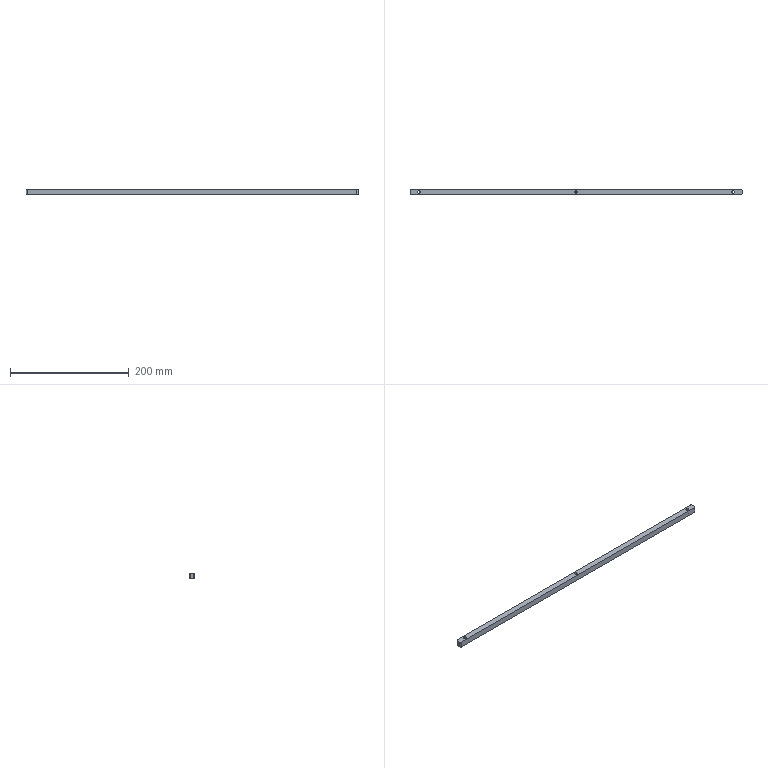Component | SolidWorks | SL010-RightStreamline-1-1_SL010-02047844SupportBar2-1-1 | 1 solid | 25 faces | box 560 x 10 x 10 mm | volume 55035 mm3 | cylinder 16 | plane 9 | commonest cylinder face diameters 8 x6 4.5 x6 4 x4 | material White POM
build123d program:
from build123d import *

# Parameters (mm, degrees)
SKETCH1_W                                       = 560
SKETCH1_H                                       = 10
BOSS_EXTRUDE1_DEPTH                             = 5
M4_HEX_SOCKET_HEAD_CAP_SCREW_CBORE1_D           = 4.5
M4_HEX_SOCKET_HEAD_CAP_SCREW_CBORE1_CBORE_D     = 8
M4_HEX_SOCKET_HEAD_CAP_SCREW_CBORE1_CBORE_DEPTH = 4.4
FILLET1_R                                       = 2


with BuildPart() as part:
    # Sketch1 → Boss-Extrude1 (new, symmetric)
    with BuildSketch(Plane.XY):
        Rectangle(SKETCH1_W, SKETCH1_H)
    extrude(amount=BOSS_EXTRUDE1_DEPTH, both=True)

    # M4 Hex Socket Head Cap Screw CBORE1 (through all)
    with Locations(Plane.XY.offset(5)):
        with Locations((-265, 0), (265, 0), (0, 0)):
            CounterBoreHole(M4_HEX_SOCKET_HEAD_CAP_SCREW_CBORE1_D / 2, M4_HEX_SOCKET_HEAD_CAP_SCREW_CBORE1_CBORE_D / 2, M4_HEX_SOCKET_HEAD_CAP_SCREW_CBORE1_CBORE_DEPTH)

    # Fillet1
    fillet1_edges = [part.edges().sort_by_distance(p)[0] for p in [
        (280, -5, 0),
        (-280, -5, 0),
        (-280, 5, 0),
        (280, 5, 0),
    ]]
    fillet(fillet1_edges, radius=FILLET1_R)


solid = part.part

# Placed as in the assembly
solid = solid.moved(Location((0, -116.404, -336.035), (180, 0, 0)))
STEP:
#1=CARTESIAN_POINT('',(10.591,-4.583,-13.253));
#2=VERTEX_POINT('',#1);
#3=CARTESIAN_POINT('',(10.276,-4.583,-13.253));
#4=VERTEX_POINT('',#3);
#5=CARTESIAN_POINT('',(10.433,-4.583,-13.253));
#6=DIRECTION('',(0.,-0.,-1.));
#7=DIRECTION('',(-1.,0.,0.));
#8=AXIS2_PLACEMENT_3D('',#5,#6,#7);
#9=CIRCLE('',#8,0.1575);
#10=EDGE_CURVE('',#2,#4,#9,.T.);
#11=ORIENTED_EDGE('',*,*,#10,.F.);
#12=CARTESIAN_POINT('',(10.591,-4.583,-13.427));
#13=VERTEX_POINT('',#12);
#14=CARTESIAN_POINT('',(10.591,-4.583,-13.427));
#15=DIRECTION('',(0.,-0.,-1.));
#16=VECTOR('',#15,39.37);
#17=LINE('',#14,#16);
#18=EDGE_CURVE('',#2,#13,#17,.T.);
#19=ORIENTED_EDGE('',*,*,#18,.T.);
#20=CARTESIAN_POINT('',(10.276,-4.583,-13.427));
#21=VERTEX_POINT('',#20);
#22=CARTESIAN_POINT('',(10.433,-4.583,-13.427));
#23=DIRECTION('',(0.,-0.,-1.));
#24=DIRECTION('',(-1.,0.,0.));
#25=AXIS2_PLACEMENT_3D('',#22,#23,#24);
#26=CIRCLE('',#25,0.1575);
#27=EDGE_CURVE('',#13,#21,#26,.T.);
#28=ORIENTED_EDGE('',*,*,#27,.T.);
#29=CARTESIAN_POINT('',(10.276,-4.583,-13.427));
#30=DIRECTION('',(0.,-0.,-1.));
#31=VECTOR('',#30,39.37);
#32=LINE('',#29,#31);
#33=EDGE_CURVE('',#4,#21,#32,.T.);
#34=ORIENTED_EDGE('',*,*,#33,.F.);
#35=EDGE_LOOP('',(#11,#19,#28,#34));
#36=FACE_OUTER_BOUND('',#35,.T.);
#37=CARTESIAN_POINT('',(10.433,-4.583,-13.427));
#38=DIRECTION('',(0.,-0.,-1.));
#39=DIRECTION('',(-1.,0.,0.));
#40=AXIS2_PLACEMENT_3D('',#37,#38,#39);
#41=CYLINDRICAL_SURFACE('',#40,0.1575);
#42=ADVANCED_FACE('',(#36),#41,.F.);
#43=CARTESIAN_POINT('',(10.522,-4.583,-13.033));
#44=VERTEX_POINT('',#43);
#45=CARTESIAN_POINT('',(10.344,-4.583,-13.033));
#46=VERTEX_POINT('',#45);
#47=CARTESIAN_POINT('',(10.433,-4.583,-13.033));
#48=DIRECTION('',(0.,-0.,-1.));
#49=DIRECTION('',(-1.,0.,0.));
#50=AXIS2_PLACEMENT_3D('',#47,#48,#49);
#51=CIRCLE('',#50,0.08858);
#52=EDGE_CURVE('',#44,#46,#51,.T.);
#53=ORIENTED_EDGE('',*,*,#52,.F.);
#54=CARTESIAN_POINT('',(10.522,-4.583,-13.253));
#55=VERTEX_POINT('',#54);
#56=CARTESIAN_POINT('',(10.522,-4.583,-13.427));
#57=DIRECTION('',(0.,-0.,-1.));
#58=VECTOR('',#57,39.37);
#59=LINE('',#56,#58);
#60=EDGE_CURVE('',#44,#55,#59,.T.);
#61=ORIENTED_EDGE('',*,*,#60,.T.);
#62=CARTESIAN_POINT('',(10.344,-4.583,-13.253));
#63=VERTEX_POINT('',#62);
#64=CARTESIAN_POINT('',(10.433,-4.583,-13.253));
#65=DIRECTION('',(0.,-0.,-1.));
#66=DIRECTION('',(-1.,0.,0.));
#67=AXIS2_PLACEMENT_3D('',#64,#65,#66);
#68=CIRCLE('',#67,0.08858);
#69=EDGE_CURVE('',#55,#63,#68,.T.);
#70=ORIENTED_EDGE('',*,*,#69,.T.);
#71=CARTESIAN_POINT('',(10.344,-4.583,-13.427));
#72=DIRECTION('',(0.,-0.,-1.));
#73=VECTOR('',#72,39.37);
#74=LINE('',#71,#73);
#75=EDGE_CURVE('',#46,#63,#74,.T.);
#76=ORIENTED_EDGE('',*,*,#75,.F.);
#77=EDGE_LOOP('',(#53,#61,#70,#76));
#78=FACE_OUTER_BOUND('',#77,.T.);
#79=CARTESIAN_POINT('',(10.433,-4.583,-13.427));
#80=DIRECTION('',(0.,-0.,-1.));
#81=DIRECTION('',(-1.,0.,0.));
#82=AXIS2_PLACEMENT_3D('',#79,#80,#81);
#83=CYLINDRICAL_SURFACE('',#82,0.08858);
#84=ADVANCED_FACE('',(#78),#83,.F.);
#85=CARTESIAN_POINT('',(-10.276,-4.583,-13.253));
#86=VERTEX_POINT('',#85);
#87=CARTESIAN_POINT('',(-10.591,-4.583,-13.253));
#88=VERTEX_POINT('',#87);
#89=CARTESIAN_POINT('',(-10.433,-4.583,-13.253));
#90=DIRECTION('',(0.,-0.,-1.));
#91=DIRECTION('',(-1.,0.,0.));
#92=AXIS2_PLACEMENT_3D('',#89,#90,#91);
#93=CIRCLE('',#92,0.1575);
#94=EDGE_CURVE('',#86,#88,#93,.T.);
#95=ORIENTED_EDGE('',*,*,#94,.F.);
#96=CARTESIAN_POINT('',(-10.276,-4.583,-13.427));
#97=VERTEX_POINT('',#96);
#98=CARTESIAN_POINT('',(-10.276,-4.583,-13.427));
#99=DIRECTION('',(0.,-0.,-1.));
#100=VECTOR('',#99,39.37);
#101=LINE('',#98,#100);
#102=EDGE_CURVE('',#86,#97,#101,.T.);
#103=ORIENTED_EDGE('',*,*,#102,.T.);
#104=CARTESIAN_POINT('',(-10.591,-4.583,-13.427));
#105=VERTEX_POINT('',#104);
#106=CARTESIAN_POINT('',(-10.433,-4.583,-13.427));
#107=DIRECTION('',(0.,-0.,-1.));
#108=DIRECTION('',(-1.,0.,0.));
#109=AXIS2_PLACEMENT_3D('',#106,#107,#108);
#110=CIRCLE('',#109,0.1575);
#111=EDGE_CURVE('',#97,#105,#110,.T.);
#112=ORIENTED_EDGE('',*,*,#111,.T.);
#113=CARTESIAN_POINT('',(-10.591,-4.583,-13.427));
#114=DIRECTION('',(0.,-0.,-1.));
#115=VECTOR('',#114,39.37);
#116=LINE('',#113,#115);
#117=EDGE_CURVE('',#88,#105,#116,.T.);
#118=ORIENTED_EDGE('',*,*,#117,.F.);
#119=EDGE_LOOP('',(#95,#103,#112,#118));
#120=FACE_OUTER_BOUND('',#119,.T.);
#121=CARTESIAN_POINT('',(-10.433,-4.583,-13.427));
#122=DIRECTION('',(0.,-0.,-1.));
#123=DIRECTION('',(-1.,0.,0.));
#124=AXIS2_PLACEMENT_3D('',#121,#122,#123);
#125=CYLINDRICAL_SURFACE('',#124,0.1575);
#126=ADVANCED_FACE('',(#120),#125,.F.);
#127=CARTESIAN_POINT('',(-10.344,-4.583,-13.033));
#128=VERTEX_POINT('',#127);
#129=CARTESIAN_POINT('',(-10.522,-4.583,-13.033));
#130=VERTEX_POINT('',#129);
#131=CARTESIAN_POINT('',(-10.433,-4.583,-13.033));
#132=DIRECTION('',(0.,-0.,-1.));
#133=DIRECTION('',(-1.,0.,0.));
#134=AXIS2_PLACEMENT_3D('',#131,#132,#133);
#135=CIRCLE('',#134,0.08858);
#136=EDGE_CURVE('',#128,#130,#135,.T.);
#137=ORIENTED_EDGE('',*,*,#136,.F.);
#138=CARTESIAN_POINT('',(-10.344,-4.583,-13.253));
#139=VERTEX_POINT('',#138);
#140=CARTESIAN_POINT('',(-10.344,-4.583,-13.427));
#141=DIRECTION('',(0.,-0.,-1.));
#142=VECTOR('',#141,39.37);
#143=LINE('',#140,#142);
#144=EDGE_CURVE('',#128,#139,#143,.T.);
#145=ORIENTED_EDGE('',*,*,#144,.T.);
#146=CARTESIAN_POINT('',(-10.522,-4.583,-13.253));
#147=VERTEX_POINT('',#146);
#148=CARTESIAN_POINT('',(-10.433,-4.583,-13.253));
#149=DIRECTION('',(0.,-0.,-1.));
#150=DIRECTION('',(-1.,0.,0.));
#151=AXIS2_PLACEMENT_3D('',#148,#149,#150);
#152=CIRCLE('',#151,0.08858);
#153=EDGE_CURVE('',#139,#147,#152,.T.);
#154=ORIENTED_EDGE('',*,*,#153,.T.);
#155=CARTESIAN_POINT('',(-10.522,-4.583,-13.427));
#156=DIRECTION('',(0.,-0.,-1.));
#157=VECTOR('',#156,39.37);
#158=LINE('',#155,#157);
#159=EDGE_CURVE('',#130,#147,#158,.T.);
#160=ORIENTED_EDGE('',*,*,#159,.F.);
#161=EDGE_LOOP('',(#137,#145,#154,#160));
#162=FACE_OUTER_BOUND('',#161,.T.);
#163=CARTESIAN_POINT('',(-10.433,-4.583,-13.427));
#164=DIRECTION('',(0.,-0.,-1.));
#165=DIRECTION('',(-1.,0.,0.));
#166=AXIS2_PLACEMENT_3D('',#163,#164,#165);
#167=CYLINDRICAL_SURFACE('',#166,0.08858);
#168=ADVANCED_FACE('',(#162),#167,.F.);
#169=CARTESIAN_POINT('',(0.1575,-4.583,-13.253));
#170=VERTEX_POINT('',#169);
#171=CARTESIAN_POINT('',(-0.1575,-4.583,-13.253));
#172=VERTEX_POINT('',#171);
#173=CARTESIAN_POINT('',(0.,-4.583,-13.253));
#174=DIRECTION('',(0.,-0.,-1.));
#175=DIRECTION('',(-1.,0.,0.));
#176=AXIS2_PLACEMENT_3D('',#173,#174,#175);
#177=CIRCLE('',#176,0.1575);
#178=EDGE_CURVE('',#170,#172,#177,.T.);
#179=ORIENTED_EDGE('',*,*,#178,.F.);
#180=CARTESIAN_POINT('',(0.1575,-4.583,-13.427));
#181=VERTEX_POINT('',#180);
#182=CARTESIAN_POINT('',(0.1575,-4.583,-13.427));
#183=DIRECTION('',(0.,-0.,-1.));
#184=VECTOR('',#183,39.37);
#185=LINE('',#182,#184);
#186=EDGE_CURVE('',#170,#181,#185,.T.);
#187=ORIENTED_EDGE('',*,*,#186,.T.);
#188=CARTESIAN_POINT('',(-0.1575,-4.583,-13.427));
#189=VERTEX_POINT('',#188);
#190=CARTESIAN_POINT('',(0.,-4.583,-13.427));
#191=DIRECTION('',(0.,-0.,-1.));
#192=DIRECTION('',(-1.,0.,0.));
#193=AXIS2_PLACEMENT_3D('',#190,#191,#192);
#194=CIRCLE('',#193,0.1575);
#195=EDGE_CURVE('',#181,#189,#194,.T.);
#196=ORIENTED_EDGE('',*,*,#195,.T.);
#197=CARTESIAN_POINT('',(-0.1575,-4.583,-13.427));
#198=DIRECTION('',(0.,-0.,-1.));
#199=VECTOR('',#198,39.37);
#200=LINE('',#197,#199);
#201=EDGE_CURVE('',#172,#189,#200,.T.);
#202=ORIENTED_EDGE('',*,*,#201,.F.);
#203=EDGE_LOOP('',(#179,#187,#196,#202));
#204=FACE_OUTER_BOUND('',#203,.T.);
#205=CARTESIAN_POINT('',(0.,-4.583,-13.427));
#206=DIRECTION('',(0.,-0.,-1.));
#207=DIRECTION('',(-1.,0.,0.));
#208=AXIS2_PLACEMENT_3D('',#205,#206,#207);
#209=CYLINDRICAL_SURFACE('',#208,0.1575);
#210=ADVANCED_FACE('',(#204),#209,.F.);
#211=CARTESIAN_POINT('',(0.08858,-4.583,-13.033));
#212=VERTEX_POINT('',#211);
#213=CARTESIAN_POINT('',(-0.08858,-4.583,-13.033));
#214=VERTEX_POINT('',#213);
#215=CARTESIAN_POINT('',(0.,-4.583,-13.033));
#216=DIRECTION('',(0.,-0.,-1.));
#217=DIRECTION('',(-1.,0.,0.));
#218=AXIS2_PLACEMENT_3D('',#215,#216,#217);
#219=CIRCLE('',#218,0.08858);
#220=EDGE_CURVE('',#212,#214,#219,.T.);
#221=ORIENTED_EDGE('',*,*,#220,.F.);
#222=CARTESIAN_POINT('',(0.08858,-4.583,-13.253));
#223=VERTEX_POINT('',#222);
#224=CARTESIAN_POINT('',(0.08858,-4.583,-13.427));
#225=DIRECTION('',(0.,-0.,-1.));
#226=VECTOR('',#225,39.37);
#227=LINE('',#224,#226);
#228=EDGE_CURVE('',#212,#223,#227,.T.);
#229=ORIENTED_EDGE('',*,*,#228,.T.);
#230=CARTESIAN_POINT('',(-0.08858,-4.583,-13.253));
#231=VERTEX_POINT('',#230);
#232=CARTESIAN_POINT('',(0.,-4.583,-13.253));
#233=DIRECTION('',(0.,-0.,-1.));
#234=DIRECTION('',(-1.,0.,0.));
#235=AXIS2_PLACEMENT_3D('',#232,#233,#234);
#236=CIRCLE('',#235,0.08858);
#237=EDGE_CURVE('',#223,#231,#236,.T.);
#238=ORIENTED_EDGE('',*,*,#237,.T.);
#239=CARTESIAN_POINT('',(-0.08858,-4.583,-13.427));
#240=DIRECTION('',(0.,-0.,-1.));
#241=VECTOR('',#240,39.37);
#242=LINE('',#239,#241);
#243=EDGE_CURVE('',#214,#231,#242,.T.);
#244=ORIENTED_EDGE('',*,*,#243,.F.);
#245=EDGE_LOOP('',(#221,#229,#238,#244));
#246=FACE_OUTER_BOUND('',#245,.T.);
#247=CARTESIAN_POINT('',(0.,-4.583,-13.427));
#248=DIRECTION('',(0.,-0.,-1.));
#249=DIRECTION('',(-1.,0.,0.));
#250=AXIS2_PLACEMENT_3D('',#247,#248,#249);
#251=CYLINDRICAL_SURFACE('',#250,0.08858);
#252=ADVANCED_FACE('',(#246),#251,.F.);
#253=CARTESIAN_POINT('',(-11.024,-4.701,-13.427));
#254=VERTEX_POINT('',#253);
#255=CARTESIAN_POINT('',(-11.024,-4.465,-13.427));
#256=VERTEX_POINT('',#255);
#257=CARTESIAN_POINT('',(-11.024,-4.386,-13.427));
#258=DIRECTION('',(0.,1.,-0.));
#259=VECTOR('',#258,39.37);
#260=LINE('',#257,#259);
#261=EDGE_CURVE('',#254,#256,#260,.T.);
#262=ORIENTED_EDGE('',*,*,#261,.F.);
#263=CARTESIAN_POINT('',(-11.024,-4.701,-13.033));
#264=VERTEX_POINT('',#263);
#265=CARTESIAN_POINT('',(-11.024,-4.701,-13.427));
#266=DIRECTION('',(-0.,0.,1.));
#267=VECTOR('',#266,39.37);
#268=LINE('',#265,#267);
#269=EDGE_CURVE('',#254,#264,#268,.T.);
#270=ORIENTED_EDGE('',*,*,#269,.T.);
#271=CARTESIAN_POINT('',(-11.024,-4.465,-13.033));
#272=VERTEX_POINT('',#271);
#273=CARTESIAN_POINT('',(-11.024,-4.386,-13.033));
#274=DIRECTION('',(0.,1.,-0.));
#275=VECTOR('',#274,39.37);
#276=LINE('',#273,#275);
#277=EDGE_CURVE('',#264,#272,#276,.T.);
#278=ORIENTED_EDGE('',*,*,#277,.T.);
#279=CARTESIAN_POINT('',(-11.024,-4.465,-13.427));
#280=DIRECTION('',(0.,-0.,-1.));
#281=VECTOR('',#280,39.37);
#282=LINE('',#279,#281);
#283=EDGE_CURVE('',#272,#256,#282,.T.);
#284=ORIENTED_EDGE('',*,*,#283,.T.);
#285=EDGE_LOOP('',(#262,#270,#278,#284));
#286=FACE_OUTER_BOUND('',#285,.T.);
#287=CARTESIAN_POINT('',(-11.024,-4.386,-13.427));
#288=DIRECTION('',(1.,0.,0.));
#289=DIRECTION('',(0.,-0.,-1.));
#290=AXIS2_PLACEMENT_3D('',#287,#288,#289);
#291=PLANE('',#290);
#292=ADVANCED_FACE('',(#286),#291,.F.);
#293=CARTESIAN_POINT('',(-10.945,-4.386,-13.427));
#294=VERTEX_POINT('',#293);
#295=CARTESIAN_POINT('',(10.945,-4.386,-13.427));
#296=VERTEX_POINT('',#295);
#297=CARTESIAN_POINT('',(11.024,-4.386,-13.427));
#298=DIRECTION('',(1.,0.,-0.));
#299=VECTOR('',#298,39.37);
#300=LINE('',#297,#299);
#301=EDGE_CURVE('',#294,#296,#300,.T.);
#302=ORIENTED_EDGE('',*,*,#301,.F.);
#303=CARTESIAN_POINT('',(-10.945,-4.386,-13.033));
#304=VERTEX_POINT('',#303);
#305=CARTESIAN_POINT('',(-10.945,-4.386,-13.427));
#306=DIRECTION('',(-0.,0.,1.));
#307=VECTOR('',#306,39.37);
#308=LINE('',#305,#307);
#309=EDGE_CURVE('',#294,#304,#308,.T.);
#310=ORIENTED_EDGE('',*,*,#309,.T.);
#311=CARTESIAN_POINT('',(10.945,-4.386,-13.033));
#312=VERTEX_POINT('',#311);
#313=CARTESIAN_POINT('',(11.024,-4.386,-13.033));
#314=DIRECTION('',(1.,0.,-0.));
#315=VECTOR('',#314,39.37);
#316=LINE('',#313,#315);
#317=EDGE_CURVE('',#304,#312,#316,.T.);
#318=ORIENTED_EDGE('',*,*,#317,.T.);
#319=CARTESIAN_POINT('',(10.945,-4.386,-13.427));
#320=DIRECTION('',(0.,-0.,-1.));
#321=VECTOR('',#320,39.37);
#322=LINE('',#319,#321);
#323=EDGE_CURVE('',#312,#296,#322,.T.);
#324=ORIENTED_EDGE('',*,*,#323,.T.);
#325=EDGE_LOOP('',(#302,#310,#318,#324));
#326=FACE_OUTER_BOUND('',#325,.T.);
#327=CARTESIAN_POINT('',(11.024,-4.386,-13.427));
#328=DIRECTION('',(-0.,-1.,0.));
#329=DIRECTION('',(-0.,0.,1.));
#330=AXIS2_PLACEMENT_3D('',#327,#328,#329);
#331=PLANE('',#330);
#332=ADVANCED_FACE('',(#326),#331,.F.);
#333=CARTESIAN_POINT('',(11.024,-4.465,-13.033));
#334=VERTEX_POINT('',#333);
#335=CARTESIAN_POINT('',(11.024,-4.701,-13.033));
#336=VERTEX_POINT('',#335);
#337=CARTESIAN_POINT('',(11.024,-4.386,-13.033));
#338=DIRECTION('',(-0.,-1.,0.));
#339=VECTOR('',#338,39.37);
#340=LINE('',#337,#339);
#341=EDGE_CURVE('',#334,#336,#340,.T.);
#342=ORIENTED_EDGE('',*,*,#341,.T.);
#343=CARTESIAN_POINT('',(11.024,-4.701,-13.427));
#344=VERTEX_POINT('',#343);
#345=CARTESIAN_POINT('',(11.024,-4.701,-13.427));
#346=DIRECTION('',(0.,-0.,-1.));
#347=VECTOR('',#346,39.37);
#348=LINE('',#345,#347);
#349=EDGE_CURVE('',#336,#344,#348,.T.);
#350=ORIENTED_EDGE('',*,*,#349,.T.);
#351=CARTESIAN_POINT('',(11.024,-4.465,-13.427));
#352=VERTEX_POINT('',#351);
#353=CARTESIAN_POINT('',(11.024,-4.386,-13.427));
#354=DIRECTION('',(-0.,-1.,0.));
#355=VECTOR('',#354,39.37);
#356=LINE('',#353,#355);
#357=EDGE_CURVE('',#352,#344,#356,.T.);
#358=ORIENTED_EDGE('',*,*,#357,.F.);
#359=CARTESIAN_POINT('',(11.024,-4.465,-13.427));
#360=DIRECTION('',(-0.,0.,1.));
#361=VECTOR('',#360,39.37);
#362=LINE('',#359,#361);
#363=EDGE_CURVE('',#352,#334,#362,.T.);
#364=ORIENTED_EDGE('',*,*,#363,.T.);
#365=EDGE_LOOP('',(#342,#350,#358,#364));
#366=FACE_OUTER_BOUND('',#365,.T.);
#367=CARTESIAN_POINT('',(11.024,-4.386,-13.427));
#368=DIRECTION('',(-1.,-0.,-0.));
#369=DIRECTION('',(-0.,0.,1.));
#370=AXIS2_PLACEMENT_3D('',#367,#368,#369);
#371=PLANE('',#370);
#372=ADVANCED_FACE('',(#366),#371,.F.);
#373=CARTESIAN_POINT('',(10.945,-4.78,-13.033));
#374=VERTEX_POINT('',#373);
#375=CARTESIAN_POINT('',(-10.945,-4.78,-13.033));
#376=VERTEX_POINT('',#375);
#377=CARTESIAN_POINT('',(11.024,-4.78,-13.033));
#378=DIRECTION('',(-1.,-0.,0.));
#379=VECTOR('',#378,39.37);
#380=LINE('',#377,#379);
#381=EDGE_CURVE('',#374,#376,#380,.T.);
#382=ORIENTED_EDGE('',*,*,#381,.T.);
#383=CARTESIAN_POINT('',(-10.945,-4.78,-13.427));
#384=VERTEX_POINT('',#383);
#385=CARTESIAN_POINT('',(-10.945,-4.78,-13.427));
#386=DIRECTION('',(0.,-0.,-1.));
#387=VECTOR('',#386,39.37);
#388=LINE('',#385,#387);
#389=EDGE_CURVE('',#376,#384,#388,.T.);
#390=ORIENTED_EDGE('',*,*,#389,.T.);
#391=CARTESIAN_POINT('',(10.945,-4.78,-13.427));
#392=VERTEX_POINT('',#391);
#393=CARTESIAN_POINT('',(11.024,-4.78,-13.427));
#394=DIRECTION('',(-1.,-0.,0.));
#395=VECTOR('',#394,39.37);
#396=LINE('',#393,#395);
#397=EDGE_CURVE('',#392,#384,#396,.T.);
#398=ORIENTED_EDGE('',*,*,#397,.F.);
#399=CARTESIAN_POINT('',(10.945,-4.78,-13.427));
#400=DIRECTION('',(-0.,0.,1.));
#401=VECTOR('',#400,39.37);
#402=LINE('',#399,#401);
#403=EDGE_CURVE('',#392,#374,#402,.T.);
#404=ORIENTED_EDGE('',*,*,#403,.T.);
#405=EDGE_LOOP('',(#382,#390,#398,#404));
#406=FACE_OUTER_BOUND('',#405,.T.);
#407=CARTESIAN_POINT('',(11.024,-4.78,-13.427));
#408=DIRECTION('',(0.,1.,-0.));
#409=DIRECTION('',(0.,-0.,-1.));
#410=AXIS2_PLACEMENT_3D('',#407,#408,#409);
#411=PLANE('',#410);
#412=ADVANCED_FACE('',(#406),#411,.F.);
#413=CARTESIAN_POINT('',(10.433,-4.583,-13.427));
#414=DIRECTION('',(0.,-0.,-1.));
#415=DIRECTION('',(-1.,0.,0.));
#416=AXIS2_PLACEMENT_3D('',#413,#414,#415);
#417=CIRCLE('',#416,0.1575);
#418=EDGE_CURVE('',#21,#13,#417,.T.);
#419=ORIENTED_EDGE('',*,*,#418,.F.);
#420=ORIENTED_EDGE('',*,*,#27,.F.);
#421=EDGE_LOOP('',(#419,#420));
#422=FACE_BOUND('',#421,.T.);
#423=CARTESIAN_POINT('',(-10.433,-4.583,-13.427));
#424=DIRECTION('',(0.,-0.,-1.));
#425=DIRECTION('',(-1.,0.,0.));
#426=AXIS2_PLACEMENT_3D('',#423,#424,#425);
#427=CIRCLE('',#426,0.1575);
#428=EDGE_CURVE('',#105,#97,#427,.T.);
#429=ORIENTED_EDGE('',*,*,#428,.F.);
#430=ORIENTED_EDGE('',*,*,#111,.F.);
#431=EDGE_LOOP('',(#429,#430));
#432=FACE_BOUND('',#431,.T.);
#433=CARTESIAN_POINT('',(0.,-4.583,-13.427));
#434=DIRECTION('',(0.,-0.,-1.));
#435=DIRECTION('',(-1.,0.,0.));
#436=AXIS2_PLACEMENT_3D('',#433,#434,#435);
#437=CIRCLE('',#436,0.1575);
#438=EDGE_CURVE('',#189,#181,#437,.T.);
#439=ORIENTED_EDGE('',*,*,#438,.F.);
#440=ORIENTED_EDGE('',*,*,#195,.F.);
#441=EDGE_LOOP('',(#439,#440));
#442=FACE_BOUND('',#441,.T.);
#443=ORIENTED_EDGE('',*,*,#397,.T.);
#444=CARTESIAN_POINT('',(-10.945,-4.701,-13.427));
#445=DIRECTION('',(0.,-0.,-1.));
#446=DIRECTION('',(-1.,0.,0.));
#447=AXIS2_PLACEMENT_3D('',#444,#445,#446);
#448=CIRCLE('',#447,0.07874);
#449=EDGE_CURVE('',#384,#254,#448,.T.);
#450=ORIENTED_EDGE('',*,*,#449,.T.);
#451=ORIENTED_EDGE('',*,*,#261,.T.);
#452=CARTESIAN_POINT('',(-10.945,-4.465,-13.427));
#453=DIRECTION('',(0.,-0.,-1.));
#454=DIRECTION('',(-1.,0.,0.));
#455=AXIS2_PLACEMENT_3D('',#452,#453,#454);
#456=CIRCLE('',#455,0.07874);
#457=EDGE_CURVE('',#256,#294,#456,.T.);
#458=ORIENTED_EDGE('',*,*,#457,.T.);
#459=ORIENTED_EDGE('',*,*,#301,.T.);
#460=CARTESIAN_POINT('',(10.945,-4.465,-13.427));
#461=DIRECTION('',(0.,-0.,-1.));
#462=DIRECTION('',(-1.,0.,0.));
#463=AXIS2_PLACEMENT_3D('',#460,#461,#462);
#464=CIRCLE('',#463,0.07874);
#465=EDGE_CURVE('',#296,#352,#464,.T.);
#466=ORIENTED_EDGE('',*,*,#465,.T.);
#467=ORIENTED_EDGE('',*,*,#357,.T.);
#468=CARTESIAN_POINT('',(10.945,-4.701,-13.427));
#469=DIRECTION('',(0.,-0.,-1.));
#470=DIRECTION('',(-1.,0.,0.));
#471=AXIS2_PLACEMENT_3D('',#468,#469,#470);
#472=CIRCLE('',#471,0.07874);
#473=EDGE_CURVE('',#344,#392,#472,.T.);
#474=ORIENTED_EDGE('',*,*,#473,.T.);
#475=EDGE_LOOP('',(#443,#450,#451,#458,#459,#466,#467,#474));
#476=FACE_OUTER_BOUND('',#475,.T.);
#477=CARTESIAN_POINT('',(0.,-4.583,-13.427));
#478=DIRECTION('',(-0.,-0.,-1.));
#479=DIRECTION('',(-1.,-0.,0.));
#480=AXIS2_PLACEMENT_3D('',#477,#478,#479);
#481=PLANE('',#480);
#482=ADVANCED_FACE('',(#422,#432,#442,#476),#481,.T.);
#483=CARTESIAN_POINT('',(10.433,-4.583,-13.033));
#484=DIRECTION('',(0.,-0.,-1.));
#485=DIRECTION('',(-1.,0.,0.));
#486=AXIS2_PLACEMENT_3D('',#483,#484,#485);
#487=CIRCLE('',#486,0.08858);
#488=EDGE_CURVE('',#46,#44,#487,.T.);
#489=ORIENTED_EDGE('',*,*,#488,.T.);
#490=ORIENTED_EDGE('',*,*,#52,.T.);
#491=EDGE_LOOP('',(#489,#490));
#492=FACE_BOUND('',#491,.T.);
#493=CARTESIAN_POINT('',(-10.433,-4.583,-13.033));
#494=DIRECTION('',(0.,-0.,-1.));
#495=DIRECTION('',(-1.,0.,0.));
#496=AXIS2_PLACEMENT_3D('',#493,#494,#495);
#497=CIRCLE('',#496,0.08858);
#498=EDGE_CURVE('',#130,#128,#497,.T.);
#499=ORIENTED_EDGE('',*,*,#498,.T.);
#500=ORIENTED_EDGE('',*,*,#136,.T.);
#501=EDGE_LOOP('',(#499,#500));
#502=FACE_BOUND('',#501,.T.);
#503=CARTESIAN_POINT('',(0.,-4.583,-13.033));
#504=DIRECTION('',(0.,-0.,-1.));
#505=DIRECTION('',(-1.,0.,0.));
#506=AXIS2_PLACEMENT_3D('',#503,#504,#505);
#507=CIRCLE('',#506,0.08858);
#508=EDGE_CURVE('',#214,#212,#507,.T.);
#509=ORIENTED_EDGE('',*,*,#508,.T.);
#510=ORIENTED_EDGE('',*,*,#220,.T.);
#511=EDGE_LOOP('',(#509,#510));
#512=FACE_BOUND('',#511,.T.);
#513=ORIENTED_EDGE('',*,*,#277,.F.);
#514=CARTESIAN_POINT('',(-10.945,-4.701,-13.033));
#515=DIRECTION('',(-0.,0.,1.));
#516=DIRECTION('',(-1.,0.,0.));
#517=AXIS2_PLACEMENT_3D('',#514,#515,#516);
#518=CIRCLE('',#517,0.07874);
#519=EDGE_CURVE('',#264,#376,#518,.T.);
#520=ORIENTED_EDGE('',*,*,#519,.T.);
#521=ORIENTED_EDGE('',*,*,#381,.F.);
#522=CARTESIAN_POINT('',(10.945,-4.701,-13.033));
#523=DIRECTION('',(-0.,0.,1.));
#524=DIRECTION('',(-1.,0.,0.));
#525=AXIS2_PLACEMENT_3D('',#522,#523,#524);
#526=CIRCLE('',#525,0.07874);
#527=EDGE_CURVE('',#374,#336,#526,.T.);
#528=ORIENTED_EDGE('',*,*,#527,.T.);
#529=ORIENTED_EDGE('',*,*,#341,.F.);
#530=CARTESIAN_POINT('',(10.945,-4.465,-13.033));
#531=DIRECTION('',(-0.,0.,1.));
#532=DIRECTION('',(-1.,0.,0.));
#533=AXIS2_PLACEMENT_3D('',#530,#531,#532);
#534=CIRCLE('',#533,0.07874);
#535=EDGE_CURVE('',#334,#312,#534,.T.);
#536=ORIENTED_EDGE('',*,*,#535,.T.);
#537=ORIENTED_EDGE('',*,*,#317,.F.);
#538=CARTESIAN_POINT('',(-10.945,-4.465,-13.033));
#539=DIRECTION('',(-0.,0.,1.));
#540=DIRECTION('',(-1.,0.,0.));
#541=AXIS2_PLACEMENT_3D('',#538,#539,#540);
#542=CIRCLE('',#541,0.07874);
#543=EDGE_CURVE('',#304,#272,#542,.T.);
#544=ORIENTED_EDGE('',*,*,#543,.T.);
#545=EDGE_LOOP('',(#513,#520,#521,#528,#529,#536,#537,#544));
#546=FACE_OUTER_BOUND('',#545,.T.);
#547=CARTESIAN_POINT('',(0.,-4.583,-13.033));
#548=DIRECTION('',(-0.,-0.,-1.));
#549=DIRECTION('',(-1.,-0.,0.));
#550=AXIS2_PLACEMENT_3D('',#547,#548,#549);
#551=PLANE('',#550);
#552=ADVANCED_FACE('',(#492,#502,#512,#546),#551,.F.);
#553=ORIENTED_EDGE('',*,*,#228,.F.);
#554=ORIENTED_EDGE('',*,*,#508,.F.);
#555=ORIENTED_EDGE('',*,*,#243,.T.);
#556=CARTESIAN_POINT('',(0.,-4.583,-13.253));
#557=DIRECTION('',(0.,-0.,-1.));
#558=DIRECTION('',(-1.,0.,0.));
#559=AXIS2_PLACEMENT_3D('',#556,#557,#558);
#560=CIRCLE('',#559,0.08858);
#561=EDGE_CURVE('',#231,#223,#560,.T.);
#562=ORIENTED_EDGE('',*,*,#561,.T.);
#563=EDGE_LOOP('',(#553,#554,#555,#562));
#564=FACE_OUTER_BOUND('',#563,.T.);
#565=CARTESIAN_POINT('',(0.,-4.583,-13.427));
#566=DIRECTION('',(0.,-0.,-1.));
#567=DIRECTION('',(-1.,0.,0.));
#568=AXIS2_PLACEMENT_3D('',#565,#566,#567);
#569=CYLINDRICAL_SURFACE('',#568,0.08858);
#570=ADVANCED_FACE('',(#564),#569,.F.);
#571=ORIENTED_EDGE('',*,*,#561,.F.);
#572=ORIENTED_EDGE('',*,*,#237,.F.);
#573=EDGE_LOOP('',(#571,#572));
#574=FACE_BOUND('',#573,.T.);
#575=CARTESIAN_POINT('',(0.,-4.583,-13.253));
#576=DIRECTION('',(0.,-0.,-1.));
#577=DIRECTION('',(-1.,0.,0.));
#578=AXIS2_PLACEMENT_3D('',#575,#576,#577);
#579=CIRCLE('',#578,0.1575);
#580=EDGE_CURVE('',#172,#170,#579,.T.);
#581=ORIENTED_EDGE('',*,*,#580,.T.);
#582=ORIENTED_EDGE('',*,*,#178,.T.);
#583=EDGE_LOOP('',(#581,#582));
#584=FACE_OUTER_BOUND('',#583,.T.);
#585=CARTESIAN_POINT('',(-0.08858,-4.583,-13.253));
#586=DIRECTION('',(0.,0.,1.));
#587=DIRECTION('',(1.,0.,-0.));
#588=AXIS2_PLACEMENT_3D('',#585,#586,#587);
#589=PLANE('',#588);
#590=ADVANCED_FACE('',(#574,#584),#589,.F.);
#591=ORIENTED_EDGE('',*,*,#186,.F.);
#592=ORIENTED_EDGE('',*,*,#580,.F.);
#593=ORIENTED_EDGE('',*,*,#201,.T.);
#594=ORIENTED_EDGE('',*,*,#438,.T.);
#595=EDGE_LOOP('',(#591,#592,#593,#594));
#596=FACE_OUTER_BOUND('',#595,.T.);
#597=CARTESIAN_POINT('',(0.,-4.583,-13.427));
#598=DIRECTION('',(0.,-0.,-1.));
#599=DIRECTION('',(-1.,0.,0.));
#600=AXIS2_PLACEMENT_3D('',#597,#598,#599);
#601=CYLINDRICAL_SURFACE('',#600,0.1575);
#602=ADVANCED_FACE('',(#596),#601,.F.);
#603=ORIENTED_EDGE('',*,*,#144,.F.);
#604=ORIENTED_EDGE('',*,*,#498,.F.);
#605=ORIENTED_EDGE('',*,*,#159,.T.);
#606=CARTESIAN_POINT('',(-10.433,-4.583,-13.253));
#607=DIRECTION('',(0.,-0.,-1.));
#608=DIRECTION('',(-1.,0.,0.));
#609=AXIS2_PLACEMENT_3D('',#606,#607,#608);
#610=CIRCLE('',#609,0.08858);
#611=EDGE_CURVE('',#147,#139,#610,.T.);
#612=ORIENTED_EDGE('',*,*,#611,.T.);
#613=EDGE_LOOP('',(#603,#604,#605,#612));
#614=FACE_OUTER_BOUND('',#613,.T.);
#615=CARTESIAN_POINT('',(-10.433,-4.583,-13.427));
#616=DIRECTION('',(0.,-0.,-1.));
#617=DIRECTION('',(-1.,0.,0.));
#618=AXIS2_PLACEMENT_3D('',#615,#616,#617);
#619=CYLINDRICAL_SURFACE('',#618,0.08858);
#620=ADVANCED_FACE('',(#614),#619,.F.);
#621=ORIENTED_EDGE('',*,*,#611,.F.);
#622=ORIENTED_EDGE('',*,*,#153,.F.);
#623=EDGE_LOOP('',(#621,#622));
#624=FACE_BOUND('',#623,.T.);
#625=CARTESIAN_POINT('',(-10.433,-4.583,-13.253));
#626=DIRECTION('',(0.,-0.,-1.));
#627=DIRECTION('',(-1.,0.,0.));
#628=AXIS2_PLACEMENT_3D('',#625,#626,#627);
#629=CIRCLE('',#628,0.1575);
#630=EDGE_CURVE('',#88,#86,#629,.T.);
#631=ORIENTED_EDGE('',*,*,#630,.T.);
#632=ORIENTED_EDGE('',*,*,#94,.T.);
#633=EDGE_LOOP('',(#631,#632));
#634=FACE_OUTER_BOUND('',#633,.T.);
#635=CARTESIAN_POINT('',(-10.522,-4.583,-13.253));
#636=DIRECTION('',(0.,0.,1.));
#637=DIRECTION('',(1.,0.,-0.));
#638=AXIS2_PLACEMENT_3D('',#635,#636,#637);
#639=PLANE('',#638);
#640=ADVANCED_FACE('',(#624,#634),#639,.F.);
#641=ORIENTED_EDGE('',*,*,#102,.F.);
#642=ORIENTED_EDGE('',*,*,#630,.F.);
#643=ORIENTED_EDGE('',*,*,#117,.T.);
#644=ORIENTED_EDGE('',*,*,#428,.T.);
#645=EDGE_LOOP('',(#641,#642,#643,#644));
#646=FACE_OUTER_BOUND('',#645,.T.);
#647=CARTESIAN_POINT('',(-10.433,-4.583,-13.427));
#648=DIRECTION('',(0.,-0.,-1.));
#649=DIRECTION('',(-1.,0.,0.));
#650=AXIS2_PLACEMENT_3D('',#647,#648,#649);
#651=CYLINDRICAL_SURFACE('',#650,0.1575);
#652=ADVANCED_FACE('',(#646),#651,.F.);
#653=ORIENTED_EDGE('',*,*,#60,.F.);
#654=ORIENTED_EDGE('',*,*,#488,.F.);
#655=ORIENTED_EDGE('',*,*,#75,.T.);
#656=CARTESIAN_POINT('',(10.433,-4.583,-13.253));
#657=DIRECTION('',(0.,-0.,-1.));
#658=DIRECTION('',(-1.,0.,0.));
#659=AXIS2_PLACEMENT_3D('',#656,#657,#658);
#660=CIRCLE('',#659,0.08858);
#661=EDGE_CURVE('',#63,#55,#660,.T.);
#662=ORIENTED_EDGE('',*,*,#661,.T.);
#663=EDGE_LOOP('',(#653,#654,#655,#662));
#664=FACE_OUTER_BOUND('',#663,.T.);
#665=CARTESIAN_POINT('',(10.433,-4.583,-13.427));
#666=DIRECTION('',(0.,-0.,-1.));
#667=DIRECTION('',(-1.,0.,0.));
#668=AXIS2_PLACEMENT_3D('',#665,#666,#667);
#669=CYLINDRICAL_SURFACE('',#668,0.08858);
#670=ADVANCED_FACE('',(#664),#669,.F.);
#671=ORIENTED_EDGE('',*,*,#661,.F.);
#672=ORIENTED_EDGE('',*,*,#69,.F.);
#673=EDGE_LOOP('',(#671,#672));
#674=FACE_BOUND('',#673,.T.);
#675=CARTESIAN_POINT('',(10.433,-4.583,-13.253));
#676=DIRECTION('',(0.,-0.,-1.));
#677=DIRECTION('',(-1.,0.,0.));
#678=AXIS2_PLACEMENT_3D('',#675,#676,#677);
#679=CIRCLE('',#678,0.1575);
#680=EDGE_CURVE('',#4,#2,#679,.T.);
#681=ORIENTED_EDGE('',*,*,#680,.T.);
#682=ORIENTED_EDGE('',*,*,#10,.T.);
#683=EDGE_LOOP('',(#681,#682));
#684=FACE_OUTER_BOUND('',#683,.T.);
#685=CARTESIAN_POINT('',(10.344,-4.583,-13.253));
#686=DIRECTION('',(0.,0.,1.));
#687=DIRECTION('',(1.,0.,-0.));
#688=AXIS2_PLACEMENT_3D('',#685,#686,#687);
#689=PLANE('',#688);
#690=ADVANCED_FACE('',(#674,#684),#689,.F.);
#691=ORIENTED_EDGE('',*,*,#18,.F.);
#692=ORIENTED_EDGE('',*,*,#680,.F.);
#693=ORIENTED_EDGE('',*,*,#33,.T.);
#694=ORIENTED_EDGE('',*,*,#418,.T.);
#695=EDGE_LOOP('',(#691,#692,#693,#694));
#696=FACE_OUTER_BOUND('',#695,.T.);
#697=CARTESIAN_POINT('',(10.433,-4.583,-13.427));
#698=DIRECTION('',(0.,-0.,-1.));
#699=DIRECTION('',(-1.,0.,0.));
#700=AXIS2_PLACEMENT_3D('',#697,#698,#699);
#701=CYLINDRICAL_SURFACE('',#700,0.1575);
#702=ADVANCED_FACE('',(#696),#701,.F.);
#703=ORIENTED_EDGE('',*,*,#449,.F.);
#704=ORIENTED_EDGE('',*,*,#389,.F.);
#705=ORIENTED_EDGE('',*,*,#519,.F.);
#706=ORIENTED_EDGE('',*,*,#269,.F.);
#707=EDGE_LOOP('',(#703,#704,#705,#706));
#708=FACE_OUTER_BOUND('',#707,.T.);
#709=CARTESIAN_POINT('',(-10.945,-4.701,-13.427));
#710=DIRECTION('',(-0.,0.,1.));
#711=DIRECTION('',(1.,0.,0.));
#712=AXIS2_PLACEMENT_3D('',#709,#710,#711);
#713=CYLINDRICAL_SURFACE('',#712,0.07874);
#714=ADVANCED_FACE('',(#708),#713,.T.);
#715=ORIENTED_EDGE('',*,*,#457,.F.);
#716=ORIENTED_EDGE('',*,*,#283,.F.);
#717=ORIENTED_EDGE('',*,*,#543,.F.);
#718=ORIENTED_EDGE('',*,*,#309,.F.);
#719=EDGE_LOOP('',(#715,#716,#717,#718));
#720=FACE_OUTER_BOUND('',#719,.T.);
#721=CARTESIAN_POINT('',(-10.945,-4.465,-13.427));
#722=DIRECTION('',(-0.,0.,1.));
#723=DIRECTION('',(1.,0.,0.));
#724=AXIS2_PLACEMENT_3D('',#721,#722,#723);
#725=CYLINDRICAL_SURFACE('',#724,0.07874);
#726=ADVANCED_FACE('',(#720),#725,.T.);
#727=ORIENTED_EDGE('',*,*,#473,.F.);
#728=ORIENTED_EDGE('',*,*,#349,.F.);
#729=ORIENTED_EDGE('',*,*,#527,.F.);
#730=ORIENTED_EDGE('',*,*,#403,.F.);
#731=EDGE_LOOP('',(#727,#728,#729,#730));
#732=FACE_OUTER_BOUND('',#731,.T.);
#733=CARTESIAN_POINT('',(10.945,-4.701,-13.427));
#734=DIRECTION('',(-0.,0.,1.));
#735=DIRECTION('',(1.,0.,0.));
#736=AXIS2_PLACEMENT_3D('',#733,#734,#735);
#737=CYLINDRICAL_SURFACE('',#736,0.07874);
#738=ADVANCED_FACE('',(#732),#737,.T.);
#739=ORIENTED_EDGE('',*,*,#465,.F.);
#740=ORIENTED_EDGE('',*,*,#323,.F.);
#741=ORIENTED_EDGE('',*,*,#535,.F.);
#742=ORIENTED_EDGE('',*,*,#363,.F.);
#743=EDGE_LOOP('',(#739,#740,#741,#742));
#744=FACE_OUTER_BOUND('',#743,.T.);
#745=CARTESIAN_POINT('',(10.945,-4.465,-13.427));
#746=DIRECTION('',(-0.,0.,1.));
#747=DIRECTION('',(1.,0.,0.));
#748=AXIS2_PLACEMENT_3D('',#745,#746,#747);
#749=CYLINDRICAL_SURFACE('',#748,0.07874);
#750=ADVANCED_FACE('',(#744),#749,.T.);
#751=CLOSED_SHELL('',(#42,#84,#126,#168,#210,#252,#292,#332,#372,#412,#482,#552,#570,#590,#602,#620,#640,#652,#670,#690,#702,#714,#726,#738,#750));
#752=MANIFOLD_SOLID_BREP('',#751);
#753=CARTESIAN_POINT('',(0.,0.,0.));
#754=DIRECTION('',(0.,0.,1.));
#755=DIRECTION('',(1.,0.,0.));
#756=AXIS2_PLACEMENT_3D('',#753,#754,#755);
#757=(LENGTH_UNIT()NAMED_UNIT(*)SI_UNIT($,.METRE.));
#758=LENGTH_MEASURE_WITH_UNIT(LENGTH_MEASURE(0.0254),#757);
#759=DIMENSIONAL_EXPONENTS(1.,0.,0.,0.,0.,0.,0.);
#760=(CONVERSION_BASED_UNIT('',#758)LENGTH_UNIT()NAMED_UNIT(#759));
#761=UNCERTAINTY_MEASURE_WITH_UNIT(LENGTH_MEASURE(0.00001),#760,'','');
#762=(NAMED_UNIT(*)PLANE_ANGLE_UNIT()SI_UNIT($,.RADIAN.));
#763=(NAMED_UNIT(*)SI_UNIT($,.STERADIAN.)SOLID_ANGLE_UNIT());
#764=(GEOMETRIC_REPRESENTATION_CONTEXT(3)GLOBAL_UNCERTAINTY_ASSIGNED_CONTEXT((#761))GLOBAL_UNIT_ASSIGNED_CONTEXT((#760,#762,#763))REPRESENTATION_CONTEXT('',''));
#765=ADVANCED_BREP_SHAPE_REPRESENTATION('',(#752,#756),#764);
#766=COLOUR_RGB('',0.7922,0.8196,0.9333);
#767=FILL_AREA_STYLE_COLOUR('',#766);
#768=FILL_AREA_STYLE('',(#767));
#769=SURFACE_STYLE_FILL_AREA(#768);
#770=SURFACE_SIDE_STYLE('',(#769));
#771=SURFACE_STYLE_USAGE(.BOTH.,#770);
#772=PRESENTATION_STYLE_ASSIGNMENT((#771));
#773=STYLED_ITEM('',(#772),#752);
#774=PRESENTATION_LAYER_ASSIGNMENT('','',(#773));
#775=(LENGTH_UNIT()NAMED_UNIT(*)SI_UNIT($,.METRE.));
#776=LENGTH_MEASURE_WITH_UNIT(LENGTH_MEASURE(0.0254),#775);
#777=DIMENSIONAL_EXPONENTS(1.,0.,0.,0.,0.,0.,0.);
#778=(CONVERSION_BASED_UNIT('',#776)LENGTH_UNIT()NAMED_UNIT(#777));
#779=UNCERTAINTY_MEASURE_WITH_UNIT(LENGTH_MEASURE(0.00001),#778,'','');
#780=(NAMED_UNIT(*)PLANE_ANGLE_UNIT()SI_UNIT($,.RADIAN.));
#781=(NAMED_UNIT(*)SI_UNIT($,.STERADIAN.)SOLID_ANGLE_UNIT());
#782=(GEOMETRIC_REPRESENTATION_CONTEXT(3)GLOBAL_UNCERTAINTY_ASSIGNED_CONTEXT((#779))GLOBAL_UNIT_ASSIGNED_CONTEXT((#778,#780,#781))REPRESENTATION_CONTEXT('',''));
#783=MECHANICAL_DESIGN_GEOMETRIC_PRESENTATION_REPRESENTATION('',(#773),#782);